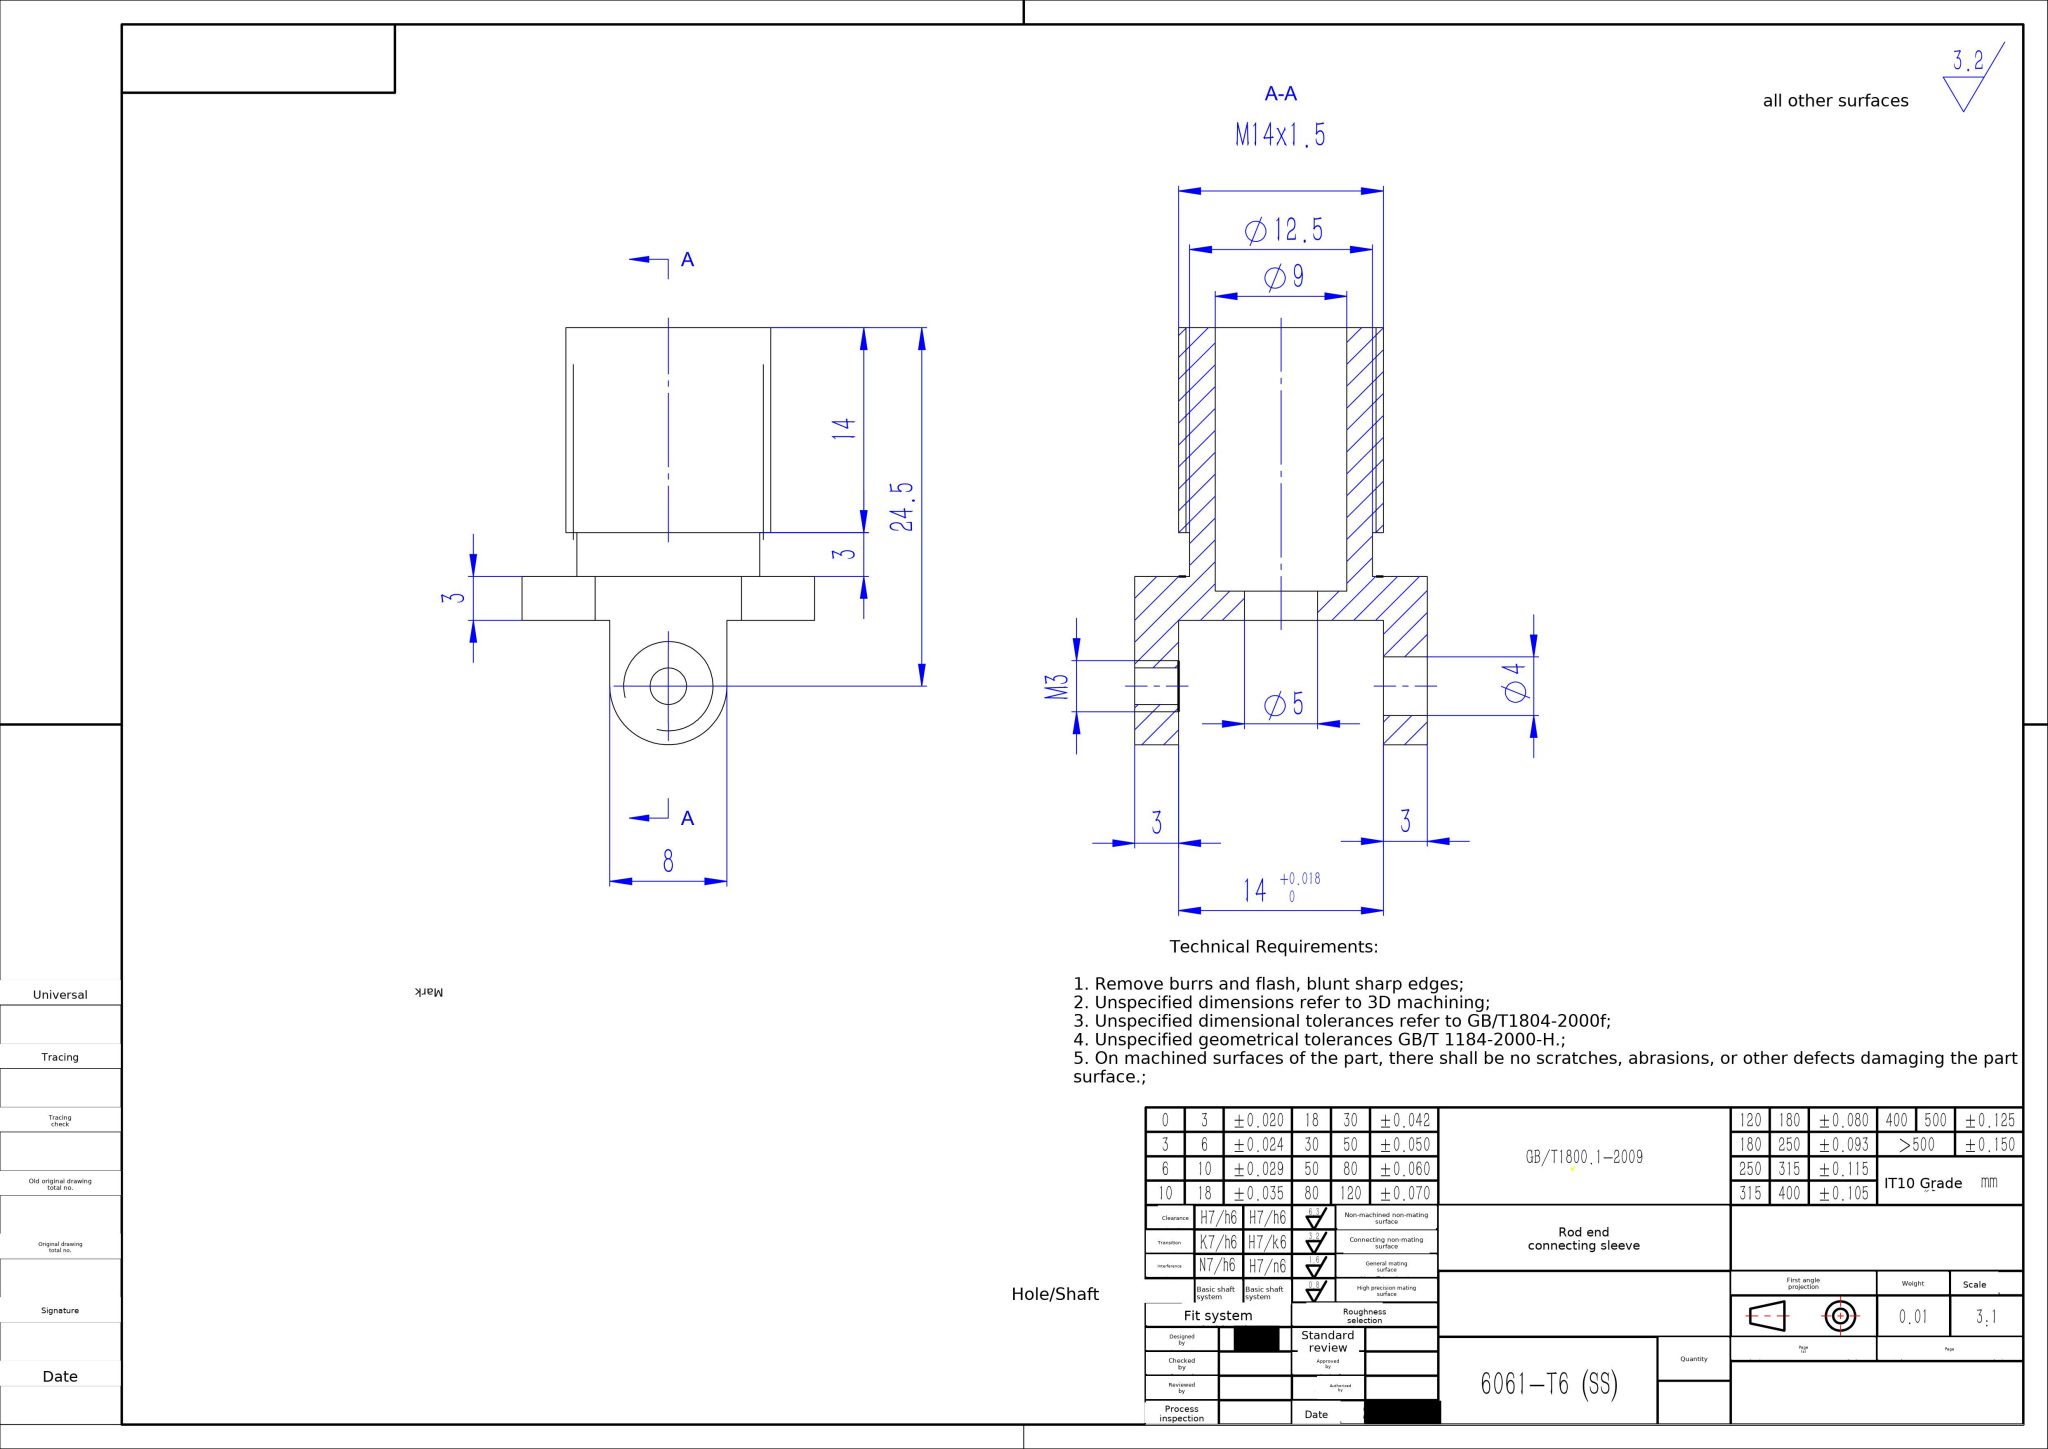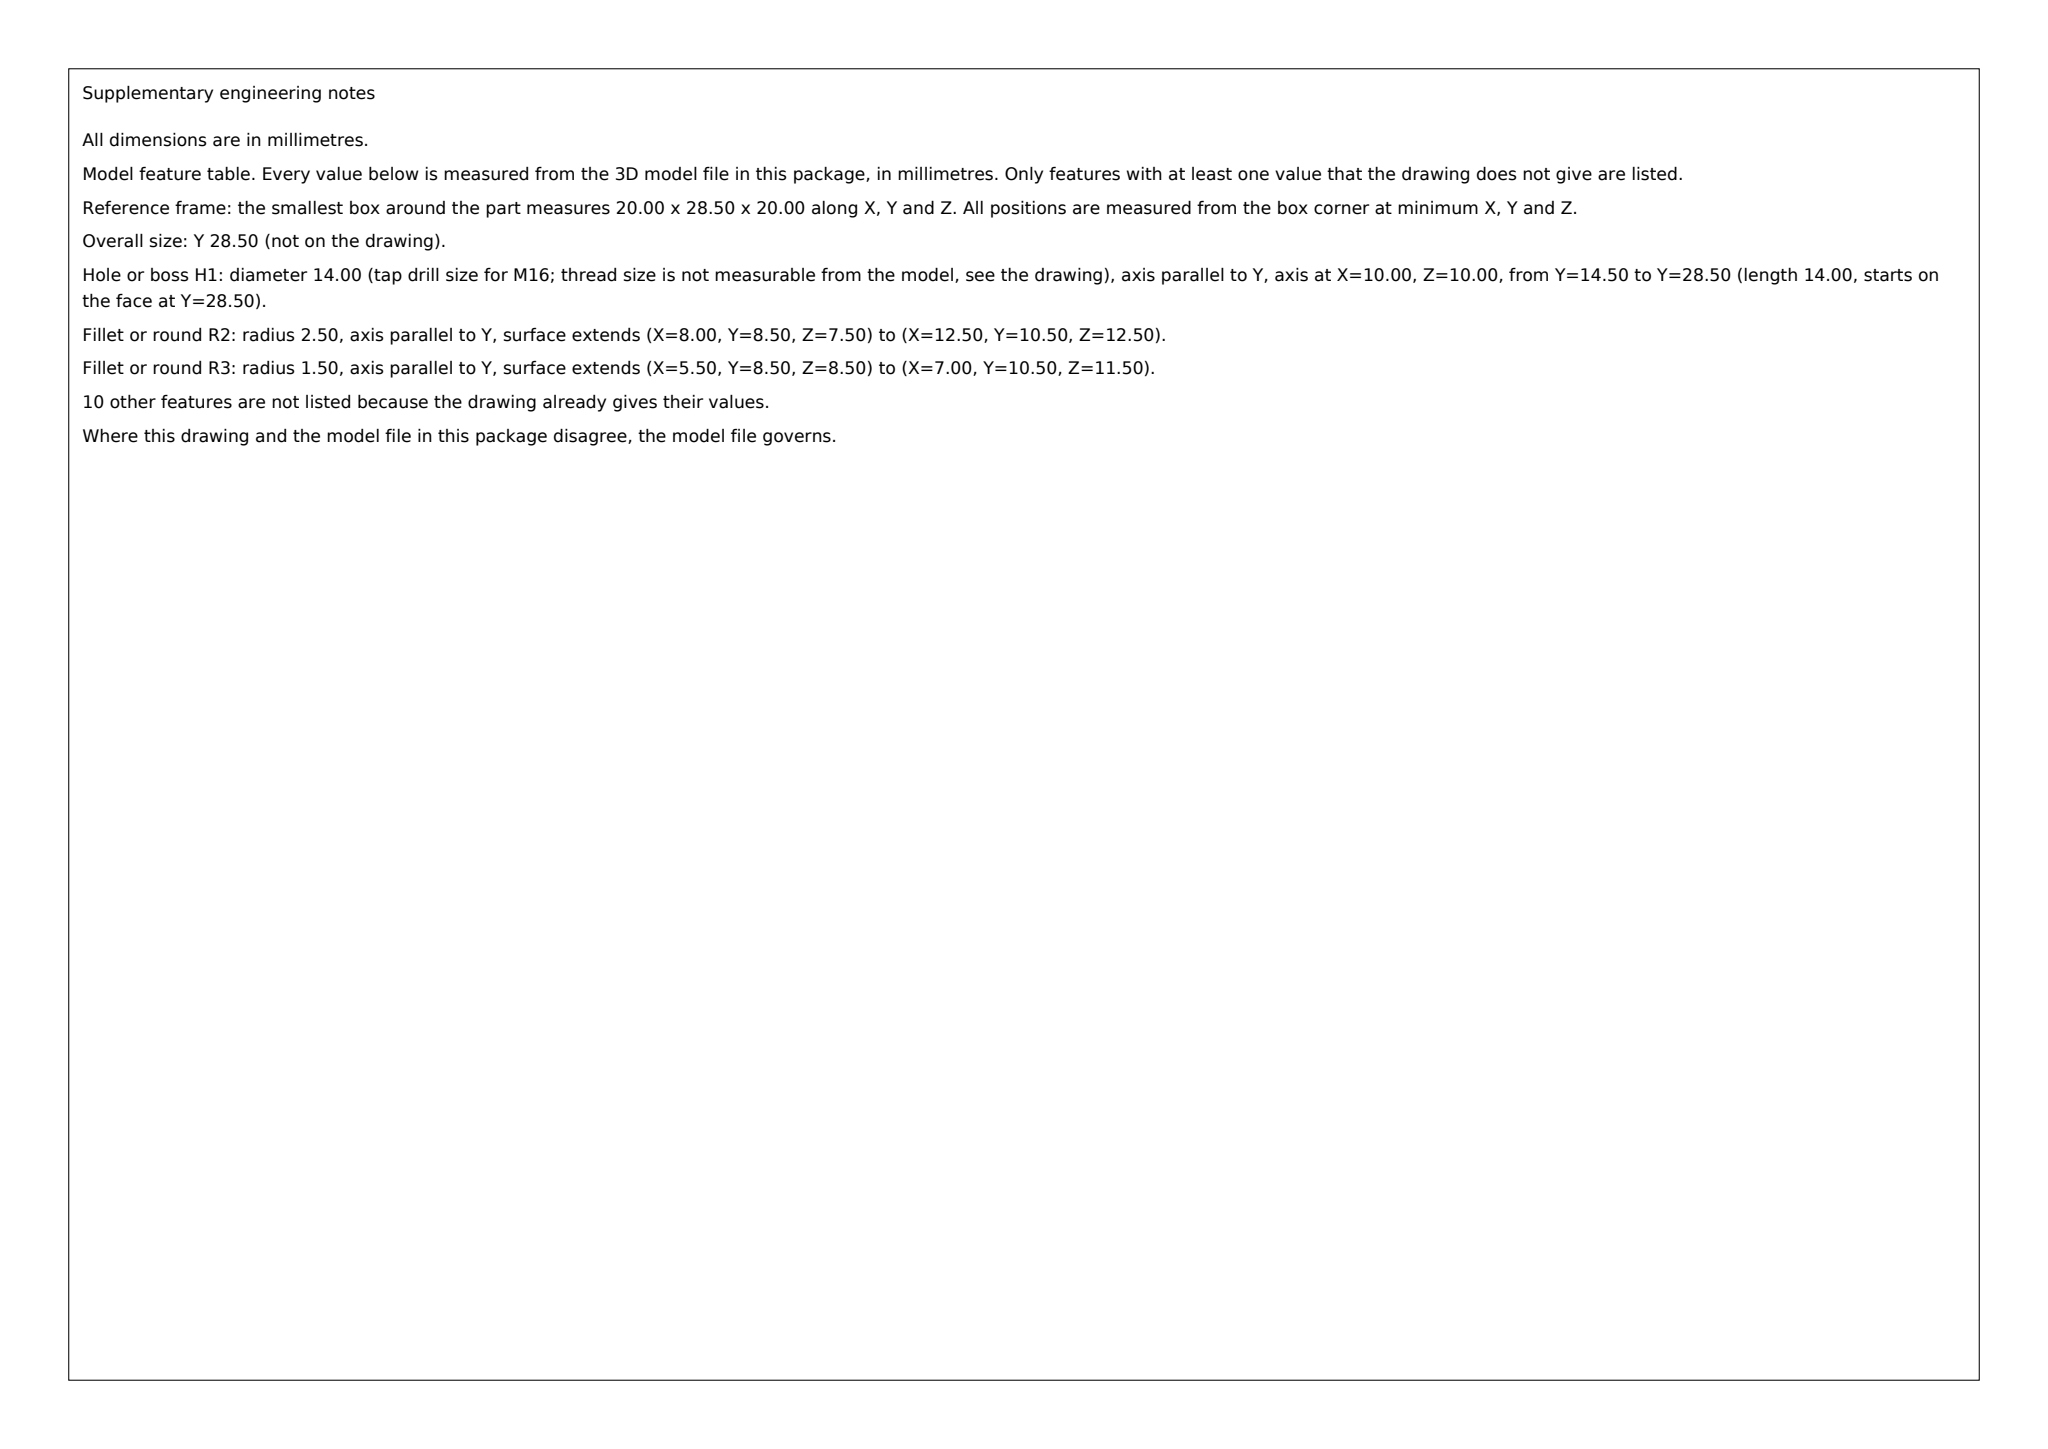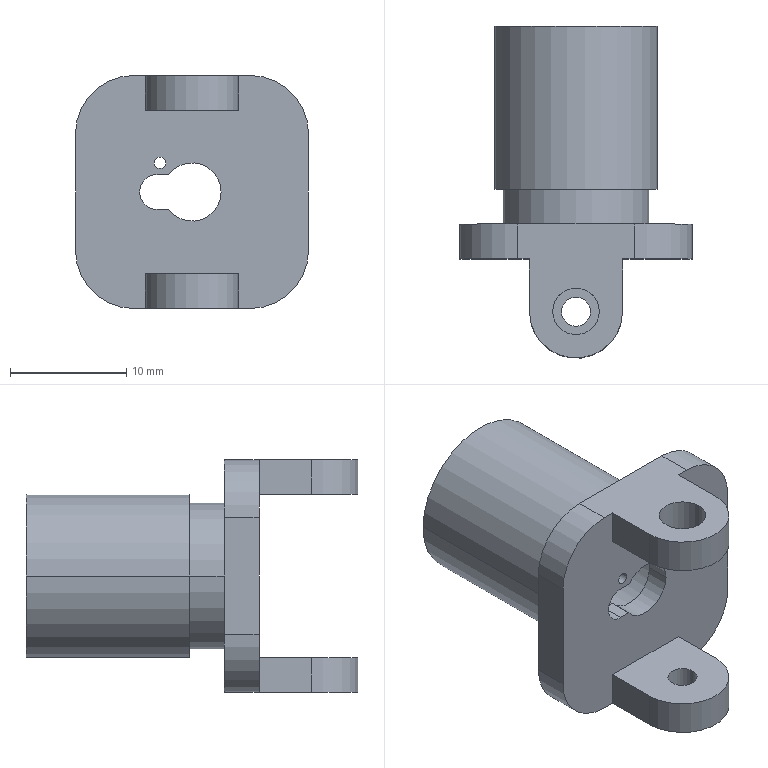Part | SolidWorks | mm | material 6061-T6 (SS) | 1 solid | 39 faces | box 20 x 28.5 x 20 mm | volume 2776 mm3 | cylinder 22 | plane 17 | commonest cylinder face diameters 10 x4 12.5 x2 3 x2 1 x2 5 x2 2.5 x2 14 x2 4 x2
build123d program:
from build123d import *

# Parameters (mm, degrees)
SKETCH1_W             = 20
SKETCH1_H             = 20
BOSS_EXTRUDE1_DEPTH   = 10
SKETCH2_R             = 2
BOSS_EXTRUDE2_DEPTH   = 10
SKETCH3_W             = 14
SKETCH3_H             = 8.5
CUT_EXTRUDE1_DEPTH    = 30.022
SKETCH4_R             = 4.5
CUT_EXTRUDE2_DEPTH    = 25.495
SKETCH5_R             = 14.142
SKETCH5_R_2           = 7
CUT_EXTRUDE3_DEPTH    = 17
FILLET1_R             = 5
SKETCH6_R             = 2
BOSS_EXTRUDE3_DEPTH   = 3
M3_TAPPED_HOLE1_D     = 2.5
M3_TAPPED_HOLE1_DEPTH = 6.749
M3_TAPPED_HOLE1_TIP   = 0.7511
SKETCH9_R             = 4.5
SKETCH9_R_2           = 2.5
BOSS_EXTRUDE4_DEPTH   = 2
SKETCH10_R            = 0.5
CUT_EXTRUDE4_DEPTH    = 5
CUT_EXTRUDE5_DEPTH    = 5
CUT_EXTRUDE6_START    = 3
SKETCH12_R            = 7
SKETCH12_R_2          = 6.25
CUT_EXTRUDE6_DEPTH    = 3


with BuildPart() as part:
    # Sketch1 → Boss-Extrude1 (new, symmetric)
    with BuildSketch(Plane.XY):
        Rectangle(SKETCH1_W, SKETCH1_H)
    extrude(amount=BOSS_EXTRUDE1_DEPTH, both=True)

    # Sketch2 → Boss-Extrude2 (add, symmetric)
    with BuildSketch(Plane.XY):
        with BuildLine():
            Line((-4, -10), (4, -10))
            Line((4, -10), (4, -14.5))
            ThreePointArc((4, -14.5), (0, -18.5), (-4, -14.5))
            Line((-4, -14.5), (-4, -10))
        make_face()
        with Locations((0, -14.5)):
            Circle(SKETCH2_R, mode=Mode.SUBTRACT)
    extrude(amount=BOSS_EXTRUDE2_DEPTH, both=True)

    # Sketch3 → Cut-Extrude1 (cut, through all)
    with BuildSketch(Plane.ZY.offset(10)):
        with Locations((0, -14.25)):
            Rectangle(SKETCH3_W, SKETCH3_H)
    extrude(amount=-CUT_EXTRUDE1_DEPTH, mode=Mode.SUBTRACT)

    # Sketch4 → Cut-Extrude2 (cut, through all)
    with BuildSketch(Plane.XZ.offset(10)):
        Circle(SKETCH4_R)
    extrude(amount=-CUT_EXTRUDE2_DEPTH, mode=Mode.SUBTRACT)

    # Sketch5 → Cut-Extrude3 (cut)
    with BuildSketch(Plane(origin=(0, 10, 0), x_dir=(1, 0, 0), z_dir=(0, 1, 0))):
        Circle(SKETCH5_R)
        with Locations(Location((0, 0, 0), (0, 0, 180))):
            Circle(SKETCH5_R_2, mode=Mode.SUBTRACT)
    extrude(amount=-CUT_EXTRUDE3_DEPTH, mode=Mode.SUBTRACT)

    # Fillet1
    fillet1_edges = [part.edges().sort_by_distance(p)[0] for p in [
        (10, -8.5, 10),
        (10, -8.5, -10),
        (-10, -8.5, -10),
        (-10, -8.5, 10),
    ]]
    fillet(fillet1_edges, radius=FILLET1_R)

    # Sketch6 → Boss-Extrude3 (add)
    with BuildSketch(Plane.XY.offset(-10)):
        with Locations(Location((0, -14.5, 0), (0, 0, 270))):
            Circle(SKETCH6_R)
    extrude(amount=BOSS_EXTRUDE3_DEPTH)

    # M3 Tapped Hole1
    with Locations(Plane(origin=(0, 0, -10), x_dir=(-1, 0, 0), z_dir=(0, 0, -1))):
        with Locations((0, -14.5)):
            Hole(M3_TAPPED_HOLE1_D / 2, depth=M3_TAPPED_HOLE1_DEPTH)
            with Locations((0, 0, -(M3_TAPPED_HOLE1_DEPTH + M3_TAPPED_HOLE1_TIP / 2))):  # 118° drill point
                Cone(0, M3_TAPPED_HOLE1_D / 2, M3_TAPPED_HOLE1_TIP, mode=Mode.SUBTRACT)

    # Sketch9 → Boss-Extrude4 (add)
    with BuildSketch(Plane.XZ.offset(10)):
        Circle(SKETCH9_R)
        Circle(SKETCH9_R_2, mode=Mode.SUBTRACT)
    extrude(amount=-BOSS_EXTRUDE4_DEPTH)

    # Sketch10 → Cut-Extrude4 (cut)
    with BuildSketch(Plane.XZ.offset(10)):
        with Locations((-2.75, 2.5)):
            Circle(SKETCH10_R)
    extrude(amount=-CUT_EXTRUDE4_DEPTH, mode=Mode.SUBTRACT)

    # Sketch11 → Cut-Extrude5 (cut)
    with BuildSketch(Plane(origin=(0, -8, 0), x_dir=(1, 0, 0), z_dir=(0, 1, 0))):
        with BuildLine():
            Line((-2, 1.5), (-3, 1.5))
            ThreePointArc((-3, 1.5), (-4.5, 0), (-3, -1.5))
            Line((-3, -1.5), (-2, -1.5))
            Line((-2, -1.5), (-2, 1.5))
        make_face()
    extrude(amount=-CUT_EXTRUDE5_DEPTH, mode=Mode.SUBTRACT)

    # Sketch12 → Cut-Extrude6 (cut)
    with BuildSketch(Plane(origin=(0, -7, 0), x_dir=(1, 0, 0), z_dir=(0, 1, 0)).offset(CUT_EXTRUDE6_START)):
        with Locations(Location((0, 0, 0), (0, 0, 180))):
            Circle(SKETCH12_R)
        with Locations(Location((0, 0, 0), (0, 0, 180))):
            Circle(SKETCH12_R_2, mode=Mode.SUBTRACT)
    extrude(amount=-CUT_EXTRUDE6_DEPTH, mode=Mode.SUBTRACT)


solid = part.part